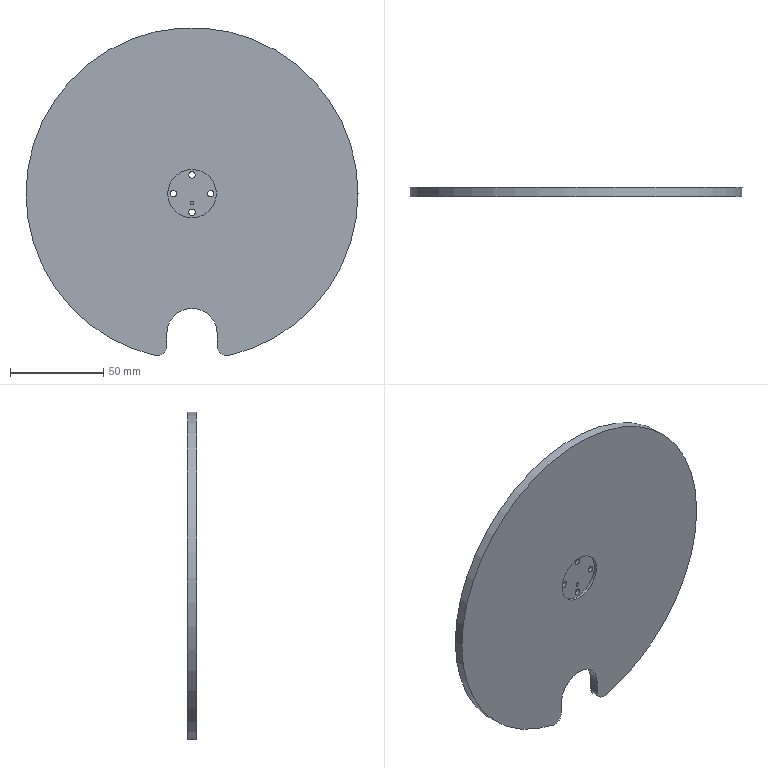CAM job | Mastercam | mm | 7 operations | part box 178 x 5 x 175.94
1. 2D High Speed (2D Area Mill) | 6 - 6 平铣刀
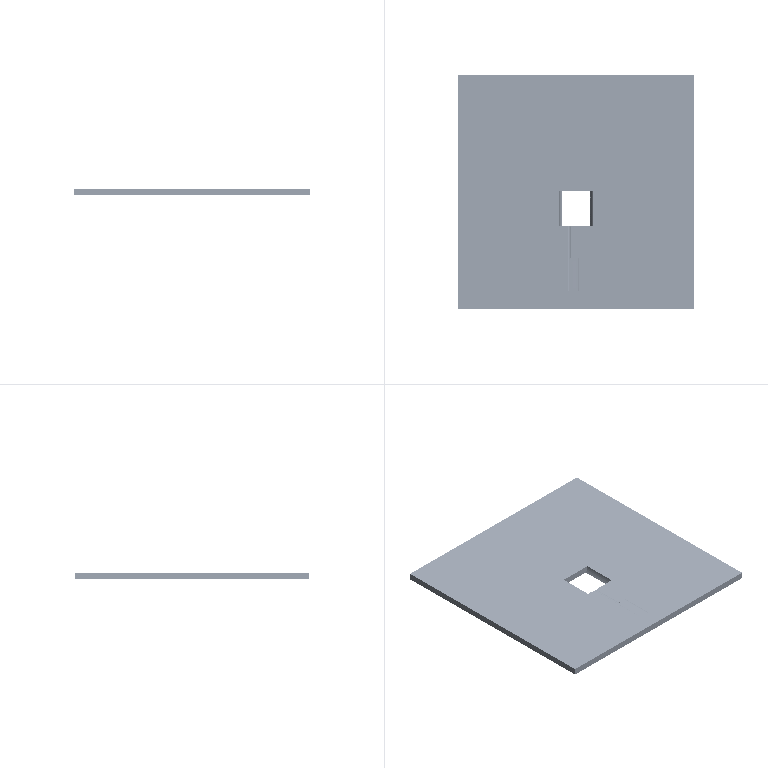2. Contour (2D) | 6 - 6 平铣刀
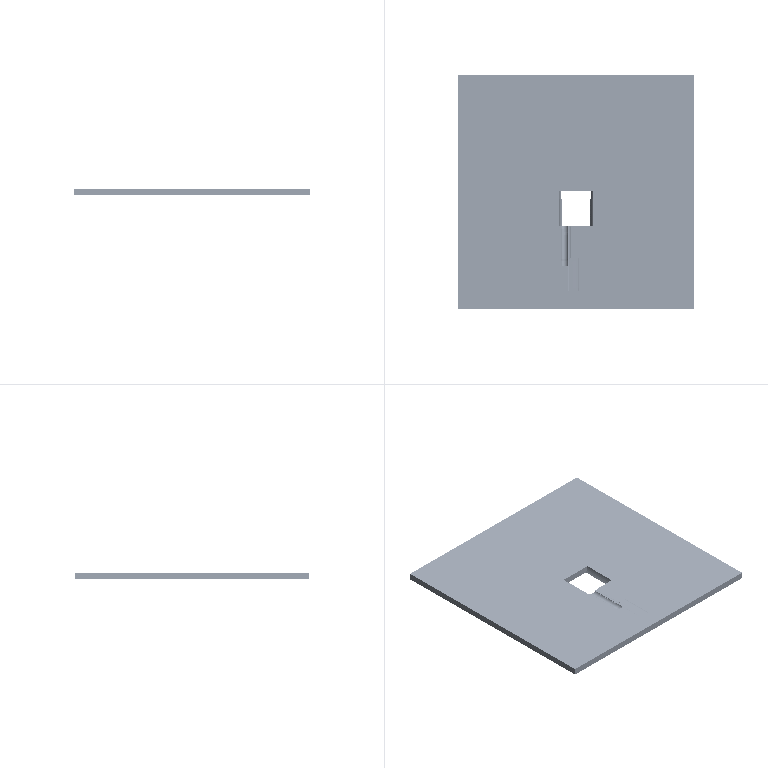3. Contour (Ramp) | 3 - 3 平铣刀
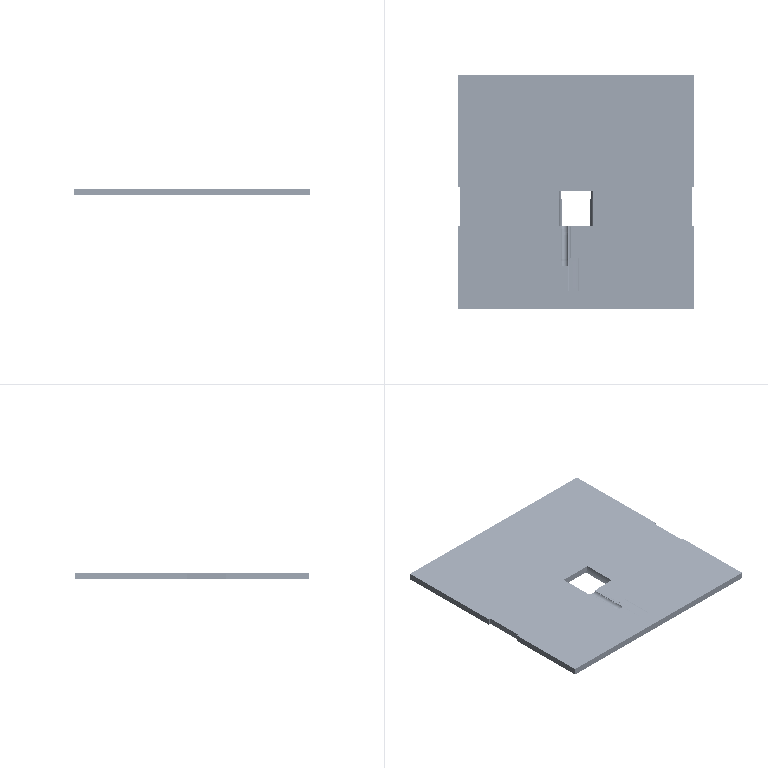4. Contour (2D) | 3 - 3 平铣刀
5. Drill/Counterbore | 7 - 4 倒角刀
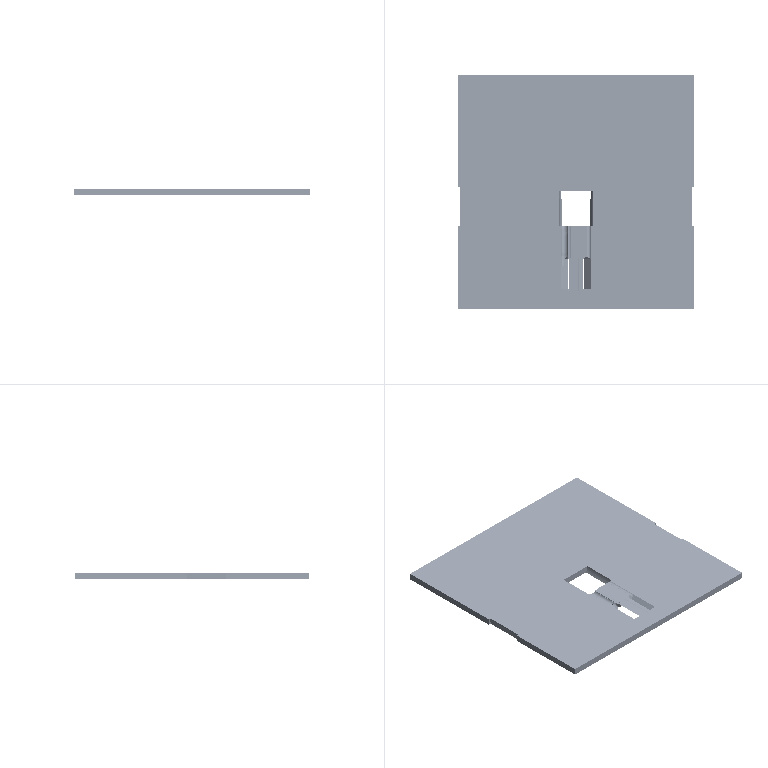6. Contour (2D chamfer) | 7 - 4 倒角刀
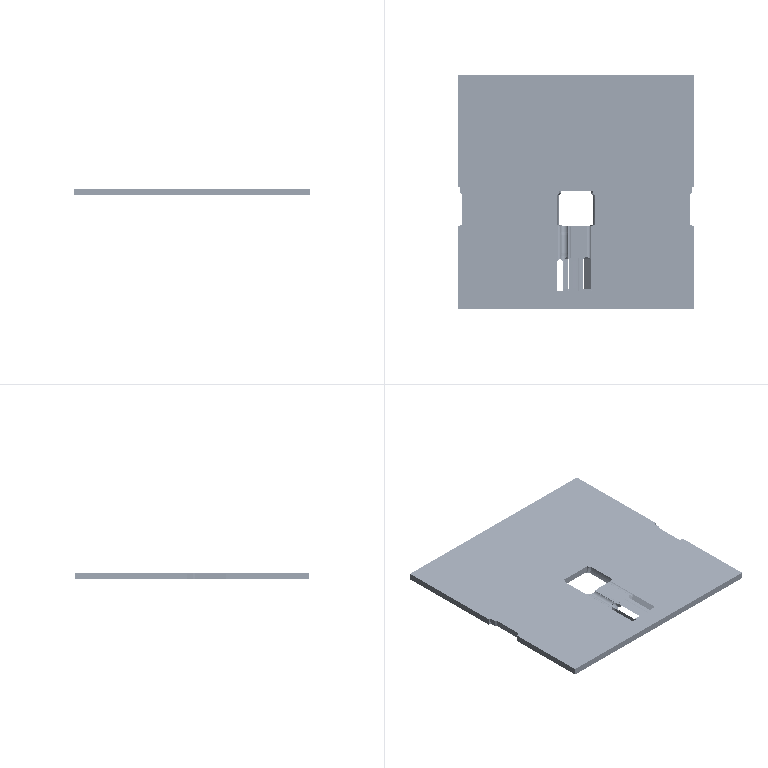7. Contour (Ramp) | 1 - 1 平铣刀